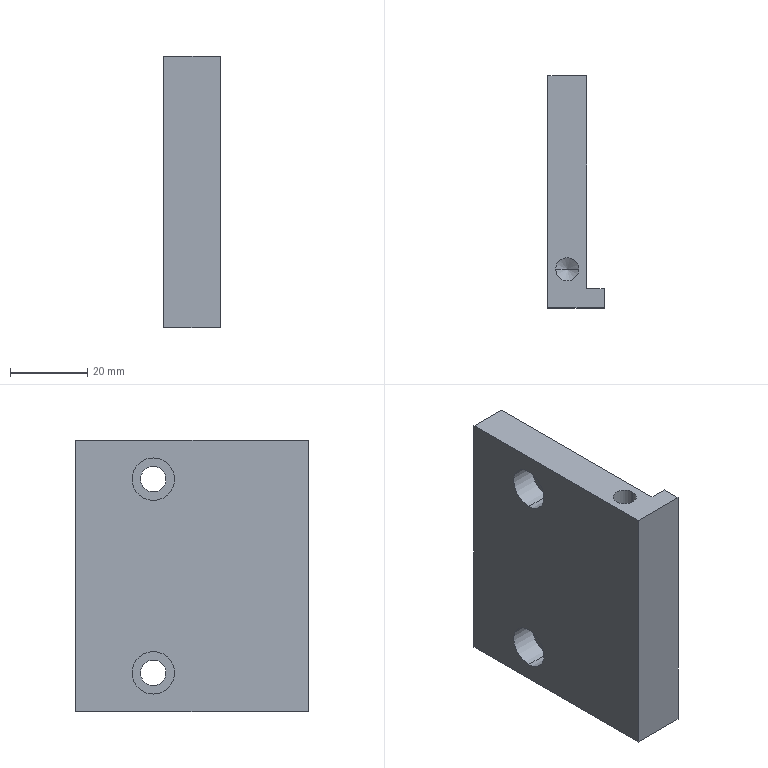Component | SolidWorks | CTM-T-12-AG-03-2 | 1 solid | 26 faces | box 14.5 x 60 x 70 mm | volume 41068 mm3 | cylinder 12 | plane 10 | cone 4 | commonest cylinder face diameters 11 x4 6.6 x4 6 x4 | material Q235A
build123d program:
from build123d import *

# Parameters (mm, degrees)
BOSS_EXTRUDE1_DEPTH                                  = 70
M6_TAPPED_HOLE1_D                                    = 6
M6_TAPPED_HOLE1_DEPTH                                = 17
M6_TAPPED_HOLE1_TIP                                  = 1.803
M6_TAPPED_HOLE2_D                                    = 6
M6_TAPPED_HOLE2_DEPTH                                = 17
M6_TAPPED_HOLE2_TIP                                  = 1.803
HOLE_SIZE_ACCORDING_TO_THE_TYPE_OF_HEXAG_D           = 6.6
HOLE_SIZE_ACCORDING_TO_THE_TYPE_OF_HEXAG_CBORE_D     = 11
HOLE_SIZE_ACCORDING_TO_THE_TYPE_OF_HEXAG_CBORE_DEPTH = 6.8


with BuildPart() as part:
    # Sketch1 → Boss-Extrude1 (new body)
    with BuildSketch(Plane.XY):
        Polygon((14.5, -5), (10, -5), (10, -60), (0, -60), (0, 0), (14.5, 0), align=None)
    extrude(amount=BOSS_EXTRUDE1_DEPTH)

    # M6 Tapped Hole1
    with Locations(Plane(origin=(0, 0, 0), x_dir=(-1, 0, 0), z_dir=(0, 0, -1))):
        with Locations((-5, -10)):
            Hole(M6_TAPPED_HOLE1_D / 2, depth=M6_TAPPED_HOLE1_DEPTH)
            with Locations((0, 0, -(M6_TAPPED_HOLE1_DEPTH + M6_TAPPED_HOLE1_TIP / 2))):  # 118° drill point
                Cone(0, M6_TAPPED_HOLE1_D / 2, M6_TAPPED_HOLE1_TIP, mode=Mode.SUBTRACT)

    # M6 Tapped Hole2
    with Locations(Plane.XY.offset(70)):
        with Locations((5, -10)):
            Hole(M6_TAPPED_HOLE2_D / 2, depth=M6_TAPPED_HOLE2_DEPTH)
            with Locations((0, 0, -(M6_TAPPED_HOLE2_DEPTH + M6_TAPPED_HOLE2_TIP / 2))):  # 118° drill point
                Cone(0, M6_TAPPED_HOLE2_D / 2, M6_TAPPED_HOLE2_TIP, mode=Mode.SUBTRACT)

    # Hole Size according to the type of Hexag (through all)
    with Locations(Plane.ZY):
        with Locations((10, -40), (60, -40)):
            CounterBoreHole(HOLE_SIZE_ACCORDING_TO_THE_TYPE_OF_HEXAG_D / 2, HOLE_SIZE_ACCORDING_TO_THE_TYPE_OF_HEXAG_CBORE_D / 2, HOLE_SIZE_ACCORDING_TO_THE_TYPE_OF_HEXAG_CBORE_DEPTH)


solid = part.part

# Placed as in the assembly
solid = solid.moved(Location((0.4, -290, 70), (180, 0, 0)))
STEP:
#1=COLOUR_RGB('',0.7922,0.8196,0.9333);
#2=FILL_AREA_STYLE_COLOUR('',#1);
#3=FILL_AREA_STYLE('',(#2));
#4=SURFACE_STYLE_FILL_AREA(#3);
#5=SURFACE_SIDE_STYLE('',(#4));
#6=SURFACE_STYLE_USAGE(.BOTH.,#5);
#7=PRESENTATION_STYLE_ASSIGNMENT((#6));
#8=CARTESIAN_POINT('',(0.2835,-9.843,2.579));
#9=VERTEX_POINT('',#8);
#10=CARTESIAN_POINT('',(0.2835,-9.843,2.146));
#11=VERTEX_POINT('',#10);
#12=CARTESIAN_POINT('',(0.2835,-9.843,2.362));
#13=DIRECTION('',(-1.,-0.,-0.));
#14=DIRECTION('',(0.,0.,-1.));
#15=AXIS2_PLACEMENT_3D('',#12,#13,#14);
#16=CIRCLE('',#15,0.2165);
#17=EDGE_CURVE('',#9,#11,#16,.T.);
#18=ORIENTED_EDGE('',*,*,#17,.F.);
#19=CARTESIAN_POINT('',(0.01575,-9.843,2.579));
#20=VERTEX_POINT('',#19);
#21=CARTESIAN_POINT('',(0.01575,-9.843,2.579));
#22=DIRECTION('',(-1.,-0.,-0.));
#23=VECTOR('',#22,39.37);
#24=LINE('',#21,#23);
#25=EDGE_CURVE('',#9,#20,#24,.T.);
#26=ORIENTED_EDGE('',*,*,#25,.T.);
#27=CARTESIAN_POINT('',(0.01575,-9.843,2.146));
#28=VERTEX_POINT('',#27);
#29=CARTESIAN_POINT('',(0.01575,-9.843,2.362));
#30=DIRECTION('',(-1.,-0.,-0.));
#31=DIRECTION('',(0.,0.,-1.));
#32=AXIS2_PLACEMENT_3D('',#29,#30,#31);
#33=CIRCLE('',#32,0.2165);
#34=EDGE_CURVE('',#20,#28,#33,.T.);
#35=ORIENTED_EDGE('',*,*,#34,.T.);
#36=CARTESIAN_POINT('',(0.01575,-9.843,2.146));
#37=DIRECTION('',(-1.,-0.,-0.));
#38=VECTOR('',#37,39.37);
#39=LINE('',#36,#38);
#40=EDGE_CURVE('',#11,#28,#39,.T.);
#41=ORIENTED_EDGE('',*,*,#40,.F.);
#42=EDGE_LOOP('',(#18,#26,#35,#41));
#43=FACE_OUTER_BOUND('',#42,.T.);
#44=CARTESIAN_POINT('',(0.01575,-9.843,2.362));
#45=DIRECTION('',(-1.,-0.,-0.));
#46=DIRECTION('',(0.,0.,-1.));
#47=AXIS2_PLACEMENT_3D('',#44,#45,#46);
#48=CYLINDRICAL_SURFACE('',#47,0.2165);
#49=ADVANCED_FACE('',(#43),#48,.F.);
#50=CARTESIAN_POINT('',(0.4094,-9.843,2.492));
#51=VERTEX_POINT('',#50);
#52=CARTESIAN_POINT('',(0.4094,-9.843,2.232));
#53=VERTEX_POINT('',#52);
#54=CARTESIAN_POINT('',(0.4094,-9.843,2.362));
#55=DIRECTION('',(-1.,-0.,-0.));
#56=DIRECTION('',(0.,1.,0.));
#57=AXIS2_PLACEMENT_3D('',#54,#55,#56);
#58=CIRCLE('',#57,0.1299);
#59=EDGE_CURVE('',#51,#53,#58,.T.);
#60=ORIENTED_EDGE('',*,*,#59,.F.);
#61=CARTESIAN_POINT('',(0.2835,-9.843,2.492));
#62=VERTEX_POINT('',#61);
#63=CARTESIAN_POINT('',(0.01575,-9.843,2.492));
#64=DIRECTION('',(-1.,-0.,-0.));
#65=VECTOR('',#64,39.37);
#66=LINE('',#63,#65);
#67=EDGE_CURVE('',#51,#62,#66,.T.);
#68=ORIENTED_EDGE('',*,*,#67,.T.);
#69=CARTESIAN_POINT('',(0.2835,-9.843,2.232));
#70=VERTEX_POINT('',#69);
#71=CARTESIAN_POINT('',(0.2835,-9.843,2.362));
#72=DIRECTION('',(-1.,-0.,-0.));
#73=DIRECTION('',(0.,0.,-1.));
#74=AXIS2_PLACEMENT_3D('',#71,#72,#73);
#75=CIRCLE('',#74,0.1299);
#76=EDGE_CURVE('',#62,#70,#75,.T.);
#77=ORIENTED_EDGE('',*,*,#76,.T.);
#78=CARTESIAN_POINT('',(0.01575,-9.843,2.232));
#79=DIRECTION('',(-1.,-0.,-0.));
#80=VECTOR('',#79,39.37);
#81=LINE('',#78,#80);
#82=EDGE_CURVE('',#53,#70,#81,.T.);
#83=ORIENTED_EDGE('',*,*,#82,.F.);
#84=EDGE_LOOP('',(#60,#68,#77,#83));
#85=FACE_OUTER_BOUND('',#84,.T.);
#86=CARTESIAN_POINT('',(0.01575,-9.843,2.362));
#87=DIRECTION('',(-1.,-0.,-0.));
#88=DIRECTION('',(0.,0.,-1.));
#89=AXIS2_PLACEMENT_3D('',#86,#87,#88);
#90=CYLINDRICAL_SURFACE('',#89,0.1299);
#91=ADVANCED_FACE('',(#85),#90,.F.);
#92=CARTESIAN_POINT('',(0.2835,-9.843,0.6102));
#93=VERTEX_POINT('',#92);
#94=CARTESIAN_POINT('',(0.2835,-9.843,0.1772));
#95=VERTEX_POINT('',#94);
#96=CARTESIAN_POINT('',(0.2835,-9.843,0.3937));
#97=DIRECTION('',(-1.,-0.,-0.));
#98=DIRECTION('',(0.,0.,-1.));
#99=AXIS2_PLACEMENT_3D('',#96,#97,#98);
#100=CIRCLE('',#99,0.2165);
#101=EDGE_CURVE('',#93,#95,#100,.T.);
#102=ORIENTED_EDGE('',*,*,#101,.F.);
#103=CARTESIAN_POINT('',(0.01575,-9.843,0.6102));
#104=VERTEX_POINT('',#103);
#105=CARTESIAN_POINT('',(0.01575,-9.843,0.6102));
#106=DIRECTION('',(-1.,-0.,-0.));
#107=VECTOR('',#106,39.37);
#108=LINE('',#105,#107);
#109=EDGE_CURVE('',#93,#104,#108,.T.);
#110=ORIENTED_EDGE('',*,*,#109,.T.);
#111=CARTESIAN_POINT('',(0.01575,-9.843,0.1772));
#112=VERTEX_POINT('',#111);
#113=CARTESIAN_POINT('',(0.01575,-9.843,0.3937));
#114=DIRECTION('',(-1.,-0.,-0.));
#115=DIRECTION('',(0.,0.,-1.));
#116=AXIS2_PLACEMENT_3D('',#113,#114,#115);
#117=CIRCLE('',#116,0.2165);
#118=EDGE_CURVE('',#104,#112,#117,.T.);
#119=ORIENTED_EDGE('',*,*,#118,.T.);
#120=CARTESIAN_POINT('',(0.01575,-9.843,0.1772));
#121=DIRECTION('',(-1.,-0.,-0.));
#122=VECTOR('',#121,39.37);
#123=LINE('',#120,#122);
#124=EDGE_CURVE('',#95,#112,#123,.T.);
#125=ORIENTED_EDGE('',*,*,#124,.F.);
#126=EDGE_LOOP('',(#102,#110,#119,#125));
#127=FACE_OUTER_BOUND('',#126,.T.);
#128=CARTESIAN_POINT('',(0.01575,-9.843,0.3937));
#129=DIRECTION('',(-1.,-0.,-0.));
#130=DIRECTION('',(0.,0.,-1.));
#131=AXIS2_PLACEMENT_3D('',#128,#129,#130);
#132=CYLINDRICAL_SURFACE('',#131,0.2165);
#133=ADVANCED_FACE('',(#127),#132,.F.);
#134=CARTESIAN_POINT('',(0.4094,-9.843,0.5236));
#135=VERTEX_POINT('',#134);
#136=CARTESIAN_POINT('',(0.4094,-9.843,0.2638));
#137=VERTEX_POINT('',#136);
#138=CARTESIAN_POINT('',(0.4094,-9.843,0.3937));
#139=DIRECTION('',(-1.,-0.,-0.));
#140=DIRECTION('',(0.,1.,-0.));
#141=AXIS2_PLACEMENT_3D('',#138,#139,#140);
#142=CIRCLE('',#141,0.1299);
#143=EDGE_CURVE('',#135,#137,#142,.T.);
#144=ORIENTED_EDGE('',*,*,#143,.F.);
#145=CARTESIAN_POINT('',(0.2835,-9.843,0.5236));
#146=VERTEX_POINT('',#145);
#147=CARTESIAN_POINT('',(0.01575,-9.843,0.5236));
#148=DIRECTION('',(-1.,-0.,-0.));
#149=VECTOR('',#148,39.37);
#150=LINE('',#147,#149);
#151=EDGE_CURVE('',#135,#146,#150,.T.);
#152=ORIENTED_EDGE('',*,*,#151,.T.);
#153=CARTESIAN_POINT('',(0.2835,-9.843,0.2638));
#154=VERTEX_POINT('',#153);
#155=CARTESIAN_POINT('',(0.2835,-9.843,0.3937));
#156=DIRECTION('',(-1.,-0.,-0.));
#157=DIRECTION('',(0.,0.,-1.));
#158=AXIS2_PLACEMENT_3D('',#155,#156,#157);
#159=CIRCLE('',#158,0.1299);
#160=EDGE_CURVE('',#146,#154,#159,.T.);
#161=ORIENTED_EDGE('',*,*,#160,.T.);
#162=CARTESIAN_POINT('',(0.01575,-9.843,0.2638));
#163=DIRECTION('',(-1.,-0.,-0.));
#164=VECTOR('',#163,39.37);
#165=LINE('',#162,#164);
#166=EDGE_CURVE('',#137,#154,#165,.T.);
#167=ORIENTED_EDGE('',*,*,#166,.F.);
#168=EDGE_LOOP('',(#144,#152,#161,#167));
#169=FACE_OUTER_BOUND('',#168,.T.);
#170=CARTESIAN_POINT('',(0.01575,-9.843,0.3937));
#171=DIRECTION('',(-1.,-0.,-0.));
#172=DIRECTION('',(0.,0.,-1.));
#173=AXIS2_PLACEMENT_3D('',#170,#171,#172);
#174=CYLINDRICAL_SURFACE('',#173,0.1299);
#175=ADVANCED_FACE('',(#169),#174,.F.);
#176=CARTESIAN_POINT('',(0.09449,-11.024,0.6693));
#177=VERTEX_POINT('',#176);
#178=CARTESIAN_POINT('',(0.3307,-11.024,0.6693));
#179=VERTEX_POINT('',#178);
#180=CARTESIAN_POINT('',(0.2126,-11.024,0.6693));
#181=DIRECTION('',(0.,-0.,-1.));
#182=DIRECTION('',(1.,0.,0.));
#183=AXIS2_PLACEMENT_3D('',#180,#181,#182);
#184=CIRCLE('',#183,0.1181);
#185=EDGE_CURVE('',#177,#179,#184,.T.);
#186=ORIENTED_EDGE('',*,*,#185,.F.);
#187=CARTESIAN_POINT('',(0.09449,-11.024,-0.));
#188=VERTEX_POINT('',#187);
#189=CARTESIAN_POINT('',(0.09449,-11.024,-0.));
#190=DIRECTION('',(0.,-0.,-1.));
#191=VECTOR('',#190,39.37);
#192=LINE('',#189,#191);
#193=EDGE_CURVE('',#177,#188,#192,.T.);
#194=ORIENTED_EDGE('',*,*,#193,.T.);
#195=CARTESIAN_POINT('',(0.3307,-11.024,-0.));
#196=VERTEX_POINT('',#195);
#197=CARTESIAN_POINT('',(0.2126,-11.024,-0.));
#198=DIRECTION('',(0.,-0.,-1.));
#199=DIRECTION('',(1.,0.,0.));
#200=AXIS2_PLACEMENT_3D('',#197,#198,#199);
#201=CIRCLE('',#200,0.1181);
#202=EDGE_CURVE('',#188,#196,#201,.T.);
#203=ORIENTED_EDGE('',*,*,#202,.T.);
#204=CARTESIAN_POINT('',(0.3307,-11.024,-0.));
#205=DIRECTION('',(0.,-0.,-1.));
#206=VECTOR('',#205,39.37);
#207=LINE('',#204,#206);
#208=EDGE_CURVE('',#179,#196,#207,.T.);
#209=ORIENTED_EDGE('',*,*,#208,.F.);
#210=EDGE_LOOP('',(#186,#194,#203,#209));
#211=FACE_OUTER_BOUND('',#210,.T.);
#212=CARTESIAN_POINT('',(0.2126,-11.024,-0.));
#213=DIRECTION('',(0.,-0.,-1.));
#214=DIRECTION('',(1.,0.,0.));
#215=AXIS2_PLACEMENT_3D('',#212,#213,#214);
#216=CYLINDRICAL_SURFACE('',#215,0.1181);
#217=ADVANCED_FACE('',(#211),#216,.F.);
#218=CARTESIAN_POINT('',(0.2126,-11.024,0.7403));
#219=VERTEX_POINT('',#218);
#220=CARTESIAN_POINT('',(0.3307,-11.024,0.6693));
#221=DIRECTION('',(0.8572,-0.,-0.515));
#222=VECTOR('',#221,39.37);
#223=LINE('',#220,#222);
#224=EDGE_CURVE('',#219,#179,#223,.T.);
#225=ORIENTED_EDGE('',*,*,#224,.F.);
#226=CARTESIAN_POINT('',(0.09449,-11.024,0.6693));
#227=DIRECTION('',(-0.8572,-0.,-0.515));
#228=VECTOR('',#227,39.37);
#229=LINE('',#226,#228);
#230=EDGE_CURVE('',#219,#177,#229,.T.);
#231=ORIENTED_EDGE('',*,*,#230,.T.);
#232=ORIENTED_EDGE('',*,*,#185,.T.);
#233=EDGE_LOOP('',(#225,#231,#232));
#234=FACE_OUTER_BOUND('',#233,.T.);
#235=CARTESIAN_POINT('',(0.2126,-11.024,0.6693));
#236=DIRECTION('',(0.,-0.,-1.));
#237=DIRECTION('',(1.,0.,0.));
#238=AXIS2_PLACEMENT_3D('',#235,#236,#237);
#239=CONICAL_SURFACE('',#238,0.1181,1.03);
#240=ADVANCED_FACE('',(#234),#239,.F.);
#241=CARTESIAN_POINT('',(0.3307,-11.024,2.087));
#242=VERTEX_POINT('',#241);
#243=CARTESIAN_POINT('',(0.09449,-11.024,2.087));
#244=VERTEX_POINT('',#243);
#245=CARTESIAN_POINT('',(0.2126,-11.024,2.087));
#246=DIRECTION('',(-0.,0.,1.));
#247=DIRECTION('',(-1.,0.,0.));
#248=AXIS2_PLACEMENT_3D('',#245,#246,#247);
#249=CIRCLE('',#248,0.1181);
#250=EDGE_CURVE('',#242,#244,#249,.T.);
#251=ORIENTED_EDGE('',*,*,#250,.F.);
#252=CARTESIAN_POINT('',(0.3307,-11.024,2.756));
#253=VERTEX_POINT('',#252);
#254=CARTESIAN_POINT('',(0.3307,-11.024,2.756));
#255=DIRECTION('',(-0.,0.,1.));
#256=VECTOR('',#255,39.37);
#257=LINE('',#254,#256);
#258=EDGE_CURVE('',#242,#253,#257,.T.);
#259=ORIENTED_EDGE('',*,*,#258,.T.);
#260=CARTESIAN_POINT('',(0.09449,-11.024,2.756));
#261=VERTEX_POINT('',#260);
#262=CARTESIAN_POINT('',(0.2126,-11.024,2.756));
#263=DIRECTION('',(-0.,0.,1.));
#264=DIRECTION('',(-1.,0.,0.));
#265=AXIS2_PLACEMENT_3D('',#262,#263,#264);
#266=CIRCLE('',#265,0.1181);
#267=EDGE_CURVE('',#253,#261,#266,.T.);
#268=ORIENTED_EDGE('',*,*,#267,.T.);
#269=CARTESIAN_POINT('',(0.09449,-11.024,2.756));
#270=DIRECTION('',(-0.,0.,1.));
#271=VECTOR('',#270,39.37);
#272=LINE('',#269,#271);
#273=EDGE_CURVE('',#244,#261,#272,.T.);
#274=ORIENTED_EDGE('',*,*,#273,.F.);
#275=EDGE_LOOP('',(#251,#259,#268,#274));
#276=FACE_OUTER_BOUND('',#275,.T.);
#277=CARTESIAN_POINT('',(0.2126,-11.024,2.756));
#278=DIRECTION('',(-0.,0.,1.));
#279=DIRECTION('',(-1.,0.,0.));
#280=AXIS2_PLACEMENT_3D('',#277,#278,#279);
#281=CYLINDRICAL_SURFACE('',#280,0.1181);
#282=ADVANCED_FACE('',(#276),#281,.F.);
#283=CARTESIAN_POINT('',(0.2126,-11.024,2.016));
#284=VERTEX_POINT('',#283);
#285=CARTESIAN_POINT('',(0.09449,-11.024,2.087));
#286=DIRECTION('',(-0.8572,0.,0.515));
#287=VECTOR('',#286,39.37);
#288=LINE('',#285,#287);
#289=EDGE_CURVE('',#284,#244,#288,.T.);
#290=ORIENTED_EDGE('',*,*,#289,.F.);
#291=CARTESIAN_POINT('',(0.3307,-11.024,2.087));
#292=DIRECTION('',(0.8572,0.,0.515));
#293=VECTOR('',#292,39.37);
#294=LINE('',#291,#293);
#295=EDGE_CURVE('',#284,#242,#294,.T.);
#296=ORIENTED_EDGE('',*,*,#295,.T.);
#297=ORIENTED_EDGE('',*,*,#250,.T.);
#298=EDGE_LOOP('',(#290,#296,#297));
#299=FACE_OUTER_BOUND('',#298,.T.);
#300=CARTESIAN_POINT('',(0.2126,-11.024,2.087));
#301=DIRECTION('',(-0.,0.,1.));
#302=DIRECTION('',(-1.,0.,0.));
#303=AXIS2_PLACEMENT_3D('',#300,#301,#302);
#304=CONICAL_SURFACE('',#303,0.1181,1.03);
#305=ADVANCED_FACE('',(#299),#304,.F.);
#306=CARTESIAN_POINT('',(0.01575,-9.843,2.362));
#307=DIRECTION('',(-1.,-0.,-0.));
#308=DIRECTION('',(0.,0.,-1.));
#309=AXIS2_PLACEMENT_3D('',#306,#307,#308);
#310=CIRCLE('',#309,0.2165);
#311=EDGE_CURVE('',#28,#20,#310,.T.);
#312=ORIENTED_EDGE('',*,*,#311,.F.);
#313=ORIENTED_EDGE('',*,*,#34,.F.);
#314=EDGE_LOOP('',(#312,#313));
#315=FACE_BOUND('',#314,.T.);
#316=CARTESIAN_POINT('',(0.01575,-9.843,0.3937));
#317=DIRECTION('',(-1.,-0.,-0.));
#318=DIRECTION('',(0.,0.,-1.));
#319=AXIS2_PLACEMENT_3D('',#316,#317,#318);
#320=CIRCLE('',#319,0.2165);
#321=EDGE_CURVE('',#112,#104,#320,.T.);
#322=ORIENTED_EDGE('',*,*,#321,.F.);
#323=ORIENTED_EDGE('',*,*,#118,.F.);
#324=EDGE_LOOP('',(#322,#323));
#325=FACE_BOUND('',#324,.T.);
#326=CARTESIAN_POINT('',(0.01575,-11.417,2.756));
#327=VERTEX_POINT('',#326);
#328=CARTESIAN_POINT('',(0.01575,-9.055,2.756));
#329=VERTEX_POINT('',#328);
#330=CARTESIAN_POINT('',(0.01575,-11.417,2.756));
#331=DIRECTION('',(-0.,1.,-0.));
#332=VECTOR('',#331,39.37);
#333=LINE('',#330,#332);
#334=EDGE_CURVE('',#327,#329,#333,.T.);
#335=ORIENTED_EDGE('',*,*,#334,.T.);
#336=CARTESIAN_POINT('',(0.01575,-9.055,-0.));
#337=VERTEX_POINT('',#336);
#338=CARTESIAN_POINT('',(0.01575,-9.055,-0.));
#339=DIRECTION('',(-0.,0.,1.));
#340=VECTOR('',#339,39.37);
#341=LINE('',#338,#340);
#342=EDGE_CURVE('',#337,#329,#341,.T.);
#343=ORIENTED_EDGE('',*,*,#342,.F.);
#344=CARTESIAN_POINT('',(0.01575,-11.417,-0.));
#345=VERTEX_POINT('',#344);
#346=CARTESIAN_POINT('',(0.01575,-11.417,-0.));
#347=DIRECTION('',(-0.,1.,-0.));
#348=VECTOR('',#347,39.37);
#349=LINE('',#346,#348);
#350=EDGE_CURVE('',#345,#337,#349,.T.);
#351=ORIENTED_EDGE('',*,*,#350,.F.);
#352=CARTESIAN_POINT('',(0.01575,-11.417,-0.));
#353=DIRECTION('',(-0.,0.,1.));
#354=VECTOR('',#353,39.37);
#355=LINE('',#352,#354);
#356=EDGE_CURVE('',#345,#327,#355,.T.);
#357=ORIENTED_EDGE('',*,*,#356,.T.);
#358=EDGE_LOOP('',(#335,#343,#351,#357));
#359=FACE_OUTER_BOUND('',#358,.T.);
#360=CARTESIAN_POINT('',(0.01575,-11.417,-0.));
#361=DIRECTION('',(1.,0.,0.));
#362=DIRECTION('',(0.,-1.,0.));
#363=AXIS2_PLACEMENT_3D('',#360,#361,#362);
#364=PLANE('',#363);
#365=ADVANCED_FACE('',(#315,#325,#359),#364,.F.);
#366=CARTESIAN_POINT('',(0.4094,-9.055,2.756));
#367=VERTEX_POINT('',#366);
#368=CARTESIAN_POINT('',(0.01575,-9.055,2.756));
#369=DIRECTION('',(1.,0.,0.));
#370=VECTOR('',#369,39.37);
#371=LINE('',#368,#370);
#372=EDGE_CURVE('',#329,#367,#371,.T.);
#373=ORIENTED_EDGE('',*,*,#372,.T.);
#374=CARTESIAN_POINT('',(0.4094,-9.055,-0.));
#375=VERTEX_POINT('',#374);
#376=CARTESIAN_POINT('',(0.4094,-9.055,-0.));
#377=DIRECTION('',(-0.,0.,1.));
#378=VECTOR('',#377,39.37);
#379=LINE('',#376,#378);
#380=EDGE_CURVE('',#375,#367,#379,.T.);
#381=ORIENTED_EDGE('',*,*,#380,.F.);
#382=CARTESIAN_POINT('',(0.01575,-9.055,-0.));
#383=DIRECTION('',(1.,0.,0.));
#384=VECTOR('',#383,39.37);
#385=LINE('',#382,#384);
#386=EDGE_CURVE('',#337,#375,#385,.T.);
#387=ORIENTED_EDGE('',*,*,#386,.F.);
#388=ORIENTED_EDGE('',*,*,#342,.T.);
#389=EDGE_LOOP('',(#373,#381,#387,#388));
#390=FACE_OUTER_BOUND('',#389,.T.);
#391=CARTESIAN_POINT('',(0.01575,-9.055,-0.));
#392=DIRECTION('',(0.,-1.,0.));
#393=DIRECTION('',(0.,-0.,-1.));
#394=AXIS2_PLACEMENT_3D('',#391,#392,#393);
#395=PLANE('',#394);
#396=ADVANCED_FACE('',(#390),#395,.F.);
#397=CARTESIAN_POINT('',(0.4094,-9.843,2.362));
#398=DIRECTION('',(-1.,-0.,-0.));
#399=DIRECTION('',(0.,1.,0.));
#400=AXIS2_PLACEMENT_3D('',#397,#398,#399);
#401=CIRCLE('',#400,0.1299);
#402=EDGE_CURVE('',#53,#51,#401,.T.);
#403=ORIENTED_EDGE('',*,*,#402,.T.);
#404=ORIENTED_EDGE('',*,*,#59,.T.);
#405=EDGE_LOOP('',(#403,#404));
#406=FACE_BOUND('',#405,.T.);
#407=CARTESIAN_POINT('',(0.4094,-9.843,0.3937));
#408=DIRECTION('',(-1.,-0.,-0.));
#409=DIRECTION('',(0.,1.,-0.));
#410=AXIS2_PLACEMENT_3D('',#407,#408,#409);
#411=CIRCLE('',#410,0.1299);
#412=EDGE_CURVE('',#137,#135,#411,.T.);
#413=ORIENTED_EDGE('',*,*,#412,.T.);
#414=ORIENTED_EDGE('',*,*,#143,.T.);
#415=EDGE_LOOP('',(#413,#414));
#416=FACE_BOUND('',#415,.T.);
#417=CARTESIAN_POINT('',(0.4094,-11.22,2.756));
#418=VERTEX_POINT('',#417);
#419=CARTESIAN_POINT('',(0.4094,-11.22,2.756));
#420=DIRECTION('',(0.,-1.,0.));
#421=VECTOR('',#420,39.37);
#422=LINE('',#419,#421);
#423=EDGE_CURVE('',#367,#418,#422,.T.);
#424=ORIENTED_EDGE('',*,*,#423,.T.);
#425=CARTESIAN_POINT('',(0.4094,-11.22,-0.));
#426=VERTEX_POINT('',#425);
#427=CARTESIAN_POINT('',(0.4094,-11.22,-0.));
#428=DIRECTION('',(-0.,0.,1.));
#429=VECTOR('',#428,39.37);
#430=LINE('',#427,#429);
#431=EDGE_CURVE('',#426,#418,#430,.T.);
#432=ORIENTED_EDGE('',*,*,#431,.F.);
#433=CARTESIAN_POINT('',(0.4094,-11.22,-0.));
#434=DIRECTION('',(0.,-1.,0.));
#435=VECTOR('',#434,39.37);
#436=LINE('',#433,#435);
#437=EDGE_CURVE('',#375,#426,#436,.T.);
#438=ORIENTED_EDGE('',*,*,#437,.F.);
#439=ORIENTED_EDGE('',*,*,#380,.T.);
#440=EDGE_LOOP('',(#424,#432,#438,#439));
#441=FACE_OUTER_BOUND('',#440,.T.);
#442=CARTESIAN_POINT('',(0.4094,-11.22,-0.));
#443=DIRECTION('',(-1.,-0.,-0.));
#444=DIRECTION('',(-0.,1.,-0.));
#445=AXIS2_PLACEMENT_3D('',#442,#443,#444);
#446=PLANE('',#445);
#447=ADVANCED_FACE('',(#406,#416,#441),#446,.F.);
#448=CARTESIAN_POINT('',(0.5866,-11.22,2.756));
#449=VERTEX_POINT('',#448);
#450=CARTESIAN_POINT('',(0.5866,-11.22,2.756));
#451=DIRECTION('',(1.,0.,0.));
#452=VECTOR('',#451,39.37);
#453=LINE('',#450,#452);
#454=EDGE_CURVE('',#418,#449,#453,.T.);
#455=ORIENTED_EDGE('',*,*,#454,.T.);
#456=CARTESIAN_POINT('',(0.5866,-11.22,-0.));
#457=VERTEX_POINT('',#456);
#458=CARTESIAN_POINT('',(0.5866,-11.22,-0.));
#459=DIRECTION('',(-0.,0.,1.));
#460=VECTOR('',#459,39.37);
#461=LINE('',#458,#460);
#462=EDGE_CURVE('',#457,#449,#461,.T.);
#463=ORIENTED_EDGE('',*,*,#462,.F.);
#464=CARTESIAN_POINT('',(0.5866,-11.22,-0.));
#465=DIRECTION('',(1.,0.,0.));
#466=VECTOR('',#465,39.37);
#467=LINE('',#464,#466);
#468=EDGE_CURVE('',#426,#457,#467,.T.);
#469=ORIENTED_EDGE('',*,*,#468,.F.);
#470=ORIENTED_EDGE('',*,*,#431,.T.);
#471=EDGE_LOOP('',(#455,#463,#469,#470));
#472=FACE_OUTER_BOUND('',#471,.T.);
#473=CARTESIAN_POINT('',(0.5866,-11.22,-0.));
#474=DIRECTION('',(0.,-1.,0.));
#475=DIRECTION('',(0.,-0.,-1.));
#476=AXIS2_PLACEMENT_3D('',#473,#474,#475);
#477=PLANE('',#476);
#478=ADVANCED_FACE('',(#472),#477,.F.);
#479=CARTESIAN_POINT('',(0.5866,-11.417,2.756));
#480=VERTEX_POINT('',#479);
#481=CARTESIAN_POINT('',(0.5866,-11.417,2.756));
#482=DIRECTION('',(0.,-1.,0.));
#483=VECTOR('',#482,39.37);
#484=LINE('',#481,#483);
#485=EDGE_CURVE('',#449,#480,#484,.T.);
#486=ORIENTED_EDGE('',*,*,#485,.T.);
#487=CARTESIAN_POINT('',(0.5866,-11.417,-0.));
#488=VERTEX_POINT('',#487);
#489=CARTESIAN_POINT('',(0.5866,-11.417,-0.));
#490=DIRECTION('',(-0.,0.,1.));
#491=VECTOR('',#490,39.37);
#492=LINE('',#489,#491);
#493=EDGE_CURVE('',#488,#480,#492,.T.);
#494=ORIENTED_EDGE('',*,*,#493,.F.);
#495=CARTESIAN_POINT('',(0.5866,-11.417,-0.));
#496=DIRECTION('',(0.,-1.,0.));
#497=VECTOR('',#496,39.37);
#498=LINE('',#495,#497);
#499=EDGE_CURVE('',#457,#488,#498,.T.);
#500=ORIENTED_EDGE('',*,*,#499,.F.);
#501=ORIENTED_EDGE('',*,*,#462,.T.);
#502=EDGE_LOOP('',(#486,#494,#500,#501));
#503=FACE_OUTER_BOUND('',#502,.T.);
#504=CARTESIAN_POINT('',(0.5866,-11.417,-0.));
#505=DIRECTION('',(-1.,-0.,-0.));
#506=DIRECTION('',(0.,-0.,-1.));
#507=AXIS2_PLACEMENT_3D('',#504,#505,#506);
#508=PLANE('',#507);
#509=ADVANCED_FACE('',(#503),#508,.F.);
#510=CARTESIAN_POINT('',(0.01575,-11.417,2.756));
#511=DIRECTION('',(-1.,-0.,-0.));
#512=VECTOR('',#511,39.37);
#513=LINE('',#510,#512);
#514=EDGE_CURVE('',#480,#327,#513,.T.);
#515=ORIENTED_EDGE('',*,*,#514,.T.);
#516=ORIENTED_EDGE('',*,*,#356,.F.);
#517=CARTESIAN_POINT('',(0.01575,-11.417,-0.));
#518=DIRECTION('',(-1.,-0.,-0.));
#519=VECTOR('',#518,39.37);
#520=LINE('',#517,#519);
#521=EDGE_CURVE('',#488,#345,#520,.T.);
#522=ORIENTED_EDGE('',*,*,#521,.F.);
#523=ORIENTED_EDGE('',*,*,#493,.T.);
#524=EDGE_LOOP('',(#515,#516,#522,#523));
#525=FACE_OUTER_BOUND('',#524,.T.);
#526=CARTESIAN_POINT('',(0.01575,-11.417,-0.));
#527=DIRECTION('',(-0.,1.,-0.));
#528=DIRECTION('',(-0.,0.,1.));
#529=AXIS2_PLACEMENT_3D('',#526,#527,#528);
#530=PLANE('',#529);
#531=ADVANCED_FACE('',(#525),#530,.F.);
#532=CARTESIAN_POINT('',(0.2126,-11.024,-0.));
#533=DIRECTION('',(0.,-0.,-1.));
#534=DIRECTION('',(1.,0.,0.));
#535=AXIS2_PLACEMENT_3D('',#532,#533,#534);
#536=CIRCLE('',#535,0.1181);
#537=EDGE_CURVE('',#196,#188,#536,.T.);
#538=ORIENTED_EDGE('',*,*,#537,.F.);
#539=ORIENTED_EDGE('',*,*,#202,.F.);
#540=EDGE_LOOP('',(#538,#539));
#541=FACE_BOUND('',#540,.T.);
#542=ORIENTED_EDGE('',*,*,#350,.T.);
#543=ORIENTED_EDGE('',*,*,#386,.T.);
#544=ORIENTED_EDGE('',*,*,#437,.T.);
#545=ORIENTED_EDGE('',*,*,#468,.T.);
#546=ORIENTED_EDGE('',*,*,#499,.T.);
#547=ORIENTED_EDGE('',*,*,#521,.T.);
#548=EDGE_LOOP('',(#542,#543,#544,#545,#546,#547));
#549=FACE_OUTER_BOUND('',#548,.T.);
#550=CARTESIAN_POINT('',(0.01575,-9.055,-0.));
#551=DIRECTION('',(0.,-0.,-1.));
#552=DIRECTION('',(1.,0.,0.));
#553=AXIS2_PLACEMENT_3D('',#550,#551,#552);
#554=PLANE('',#553);
#555=ADVANCED_FACE('',(#541,#549),#554,.T.);
#556=CARTESIAN_POINT('',(0.2126,-11.024,2.756));
#557=DIRECTION('',(-0.,0.,1.));
#558=DIRECTION('',(-1.,0.,0.));
#559=AXIS2_PLACEMENT_3D('',#556,#557,#558);
#560=CIRCLE('',#559,0.1181);
#561=EDGE_CURVE('',#261,#253,#560,.T.);
#562=ORIENTED_EDGE('',*,*,#561,.F.);
#563=ORIENTED_EDGE('',*,*,#267,.F.);
#564=EDGE_LOOP('',(#562,#563));
#565=FACE_BOUND('',#564,.T.);
#566=ORIENTED_EDGE('',*,*,#334,.F.);
#567=ORIENTED_EDGE('',*,*,#514,.F.);
#568=ORIENTED_EDGE('',*,*,#485,.F.);
#569=ORIENTED_EDGE('',*,*,#454,.F.);
#570=ORIENTED_EDGE('',*,*,#423,.F.);
#571=ORIENTED_EDGE('',*,*,#372,.F.);
#572=EDGE_LOOP('',(#566,#567,#568,#569,#570,#571));
#573=FACE_OUTER_BOUND('',#572,.T.);
#574=CARTESIAN_POINT('',(0.01575,-9.055,2.756));
#575=DIRECTION('',(0.,-0.,-1.));
#576=DIRECTION('',(1.,0.,0.));
#577=AXIS2_PLACEMENT_3D('',#574,#575,#576);
#578=PLANE('',#577);
#579=ADVANCED_FACE('',(#565,#573),#578,.F.);
#580=ORIENTED_EDGE('',*,*,#295,.F.);
#581=ORIENTED_EDGE('',*,*,#289,.T.);
#582=CARTESIAN_POINT('',(0.2126,-11.024,2.087));
#583=DIRECTION('',(-0.,0.,1.));
#584=DIRECTION('',(-1.,0.,0.));
#585=AXIS2_PLACEMENT_3D('',#582,#583,#584);
#586=CIRCLE('',#585,0.1181);
#587=EDGE_CURVE('',#244,#242,#586,.T.);
#588=ORIENTED_EDGE('',*,*,#587,.T.);
#589=EDGE_LOOP('',(#580,#581,#588));
#590=FACE_OUTER_BOUND('',#589,.T.);
#591=CARTESIAN_POINT('',(0.2126,-11.024,2.087));
#592=DIRECTION('',(-0.,0.,1.));
#593=DIRECTION('',(-1.,0.,0.));
#594=AXIS2_PLACEMENT_3D('',#591,#592,#593);
#595=CONICAL_SURFACE('',#594,0.1181,1.03);
#596=ADVANCED_FACE('',(#590),#595,.F.);
#597=ORIENTED_EDGE('',*,*,#258,.F.);
#598=ORIENTED_EDGE('',*,*,#587,.F.);
#599=ORIENTED_EDGE('',*,*,#273,.T.);
#600=ORIENTED_EDGE('',*,*,#561,.T.);
#601=EDGE_LOOP('',(#597,#598,#599,#600));
#602=FACE_OUTER_BOUND('',#601,.T.);
#603=CARTESIAN_POINT('',(0.2126,-11.024,2.756));
#604=DIRECTION('',(-0.,0.,1.));
#605=DIRECTION('',(-1.,0.,0.));
#606=AXIS2_PLACEMENT_3D('',#603,#604,#605);
#607=CYLINDRICAL_SURFACE('',#606,0.1181);
#608=ADVANCED_FACE('',(#602),#607,.F.);
#609=ORIENTED_EDGE('',*,*,#230,.F.);
#610=ORIENTED_EDGE('',*,*,#224,.T.);
#611=CARTESIAN_POINT('',(0.2126,-11.024,0.6693));
#612=DIRECTION('',(0.,-0.,-1.));
#613=DIRECTION('',(1.,0.,0.));
#614=AXIS2_PLACEMENT_3D('',#611,#612,#613);
#615=CIRCLE('',#614,0.1181);
#616=EDGE_CURVE('',#179,#177,#615,.T.);
#617=ORIENTED_EDGE('',*,*,#616,.T.);
#618=EDGE_LOOP('',(#609,#610,#617));
#619=FACE_OUTER_BOUND('',#618,.T.);
#620=CARTESIAN_POINT('',(0.2126,-11.024,0.6693));
#621=DIRECTION('',(0.,-0.,-1.));
#622=DIRECTION('',(1.,0.,0.));
#623=AXIS2_PLACEMENT_3D('',#620,#621,#622);
#624=CONICAL_SURFACE('',#623,0.1181,1.03);
#625=ADVANCED_FACE('',(#619),#624,.F.);
#626=ORIENTED_EDGE('',*,*,#193,.F.);
#627=ORIENTED_EDGE('',*,*,#616,.F.);
#628=ORIENTED_EDGE('',*,*,#208,.T.);
#629=ORIENTED_EDGE('',*,*,#537,.T.);
#630=EDGE_LOOP('',(#626,#627,#628,#629));
#631=FACE_OUTER_BOUND('',#630,.T.);
#632=CARTESIAN_POINT('',(0.2126,-11.024,-0.));
#633=DIRECTION('',(0.,-0.,-1.));
#634=DIRECTION('',(1.,0.,0.));
#635=AXIS2_PLACEMENT_3D('',#632,#633,#634);
#636=CYLINDRICAL_SURFACE('',#635,0.1181);
#637=ADVANCED_FACE('',(#631),#636,.F.);
#638=ORIENTED_EDGE('',*,*,#151,.F.);
#639=ORIENTED_EDGE('',*,*,#412,.F.);
#640=ORIENTED_EDGE('',*,*,#166,.T.);
#641=CARTESIAN_POINT('',(0.2835,-9.843,0.3937));
#642=DIRECTION('',(-1.,-0.,-0.));
#643=DIRECTION('',(0.,0.,-1.));
#644=AXIS2_PLACEMENT_3D('',#641,#642,#643);
#645=CIRCLE('',#644,0.1299);
#646=EDGE_CURVE('',#154,#146,#645,.T.);
#647=ORIENTED_EDGE('',*,*,#646,.T.);
#648=EDGE_LOOP('',(#638,#639,#640,#647));
#649=FACE_OUTER_BOUND('',#648,.T.);
#650=CARTESIAN_POINT('',(0.01575,-9.843,0.3937));
#651=DIRECTION('',(-1.,-0.,-0.));
#652=DIRECTION('',(0.,0.,-1.));
#653=AXIS2_PLACEMENT_3D('',#650,#651,#652);
#654=CYLINDRICAL_SURFACE('',#653,0.1299);
#655=ADVANCED_FACE('',(#649),#654,.F.);
#656=ORIENTED_EDGE('',*,*,#646,.F.);
#657=ORIENTED_EDGE('',*,*,#160,.F.);
#658=EDGE_LOOP('',(#656,#657));
#659=FACE_BOUND('',#658,.T.);
#660=CARTESIAN_POINT('',(0.2835,-9.843,0.3937));
#661=DIRECTION('',(-1.,-0.,-0.));
#662=DIRECTION('',(0.,0.,-1.));
#663=AXIS2_PLACEMENT_3D('',#660,#661,#662);
#664=CIRCLE('',#663,0.2165);
#665=EDGE_CURVE('',#95,#93,#664,.T.);
#666=ORIENTED_EDGE('',*,*,#665,.T.);
#667=ORIENTED_EDGE('',*,*,#101,.T.);
#668=EDGE_LOOP('',(#666,#667));
#669=FACE_OUTER_BOUND('',#668,.T.);
#670=CARTESIAN_POINT('',(0.2835,-9.972,0.3937));
#671=DIRECTION('',(1.,0.,0.));
#672=DIRECTION('',(-0.,0.,1.));
#673=AXIS2_PLACEMENT_3D('',#670,#671,#672);
#674=PLANE('',#673);
#675=ADVANCED_FACE('',(#659,#669),#674,.F.);
#676=ORIENTED_EDGE('',*,*,#109,.F.);
#677=ORIENTED_EDGE('',*,*,#665,.F.);
#678=ORIENTED_EDGE('',*,*,#124,.T.);
#679=ORIENTED_EDGE('',*,*,#321,.T.);
#680=EDGE_LOOP('',(#676,#677,#678,#679));
#681=FACE_OUTER_BOUND('',#680,.T.);
#682=CARTESIAN_POINT('',(0.01575,-9.843,0.3937));
#683=DIRECTION('',(-1.,-0.,-0.));
#684=DIRECTION('',(0.,0.,-1.));
#685=AXIS2_PLACEMENT_3D('',#682,#683,#684);
#686=CYLINDRICAL_SURFACE('',#685,0.2165);
#687=ADVANCED_FACE('',(#681),#686,.F.);
#688=ORIENTED_EDGE('',*,*,#67,.F.);
#689=ORIENTED_EDGE('',*,*,#402,.F.);
#690=ORIENTED_EDGE('',*,*,#82,.T.);
#691=CARTESIAN_POINT('',(0.2835,-9.843,2.362));
#692=DIRECTION('',(-1.,-0.,-0.));
#693=DIRECTION('',(0.,0.,-1.));
#694=AXIS2_PLACEMENT_3D('',#691,#692,#693);
#695=CIRCLE('',#694,0.1299);
#696=EDGE_CURVE('',#70,#62,#695,.T.);
#697=ORIENTED_EDGE('',*,*,#696,.T.);
#698=EDGE_LOOP('',(#688,#689,#690,#697));
#699=FACE_OUTER_BOUND('',#698,.T.);
#700=CARTESIAN_POINT('',(0.01575,-9.843,2.362));
#701=DIRECTION('',(-1.,-0.,-0.));
#702=DIRECTION('',(0.,0.,-1.));
#703=AXIS2_PLACEMENT_3D('',#700,#701,#702);
#704=CYLINDRICAL_SURFACE('',#703,0.1299);
#705=ADVANCED_FACE('',(#699),#704,.F.);
#706=ORIENTED_EDGE('',*,*,#696,.F.);
#707=ORIENTED_EDGE('',*,*,#76,.F.);
#708=EDGE_LOOP('',(#706,#707));
#709=FACE_BOUND('',#708,.T.);
#710=CARTESIAN_POINT('',(0.2835,-9.843,2.362));
#711=DIRECTION('',(-1.,-0.,-0.));
#712=DIRECTION('',(0.,0.,-1.));
#713=AXIS2_PLACEMENT_3D('',#710,#711,#712);
#714=CIRCLE('',#713,0.2165);
#715=EDGE_CURVE('',#11,#9,#714,.T.);
#716=ORIENTED_EDGE('',*,*,#715,.T.);
#717=ORIENTED_EDGE('',*,*,#17,.T.);
#718=EDGE_LOOP('',(#716,#717));
#719=FACE_OUTER_BOUND('',#718,.T.);
#720=CARTESIAN_POINT('',(0.2835,-9.972,2.362));
#721=DIRECTION('',(1.,0.,0.));
#722=DIRECTION('',(-0.,0.,1.));
#723=AXIS2_PLACEMENT_3D('',#720,#721,#722);
#724=PLANE('',#723);
#725=ADVANCED_FACE('',(#709,#719),#724,.F.);
#726=ORIENTED_EDGE('',*,*,#25,.F.);
#727=ORIENTED_EDGE('',*,*,#715,.F.);
#728=ORIENTED_EDGE('',*,*,#40,.T.);
#729=ORIENTED_EDGE('',*,*,#311,.T.);
#730=EDGE_LOOP('',(#726,#727,#728,#729));
#731=FACE_OUTER_BOUND('',#730,.T.);
#732=CARTESIAN_POINT('',(0.01575,-9.843,2.362));
#733=DIRECTION('',(-1.,-0.,-0.));
#734=DIRECTION('',(0.,0.,-1.));
#735=AXIS2_PLACEMENT_3D('',#732,#733,#734);
#736=CYLINDRICAL_SURFACE('',#735,0.2165);
#737=ADVANCED_FACE('',(#731),#736,.F.);
#738=CLOSED_SHELL('',(#49,#91,#133,#175,#217,#240,#282,#305,#365,#396,#447,#478,#509,#531,#555,#579,#596,#608,#625,#637,#655,#675,#687,#705,#725,#737));
#739=MANIFOLD_SOLID_BREP('',#738);
#740=STYLED_ITEM('',(#7),#739);
#741=PRESENTATION_LAYER_ASSIGNMENT('','',(#740));
#742=CARTESIAN_POINT('',(0.,0.,0.));
#743=DIRECTION('',(0.,0.,1.));
#744=DIRECTION('',(1.,0.,0.));
#745=AXIS2_PLACEMENT_3D('',#742,#743,#744);
#746=(LENGTH_UNIT()NAMED_UNIT(*)SI_UNIT($,.METRE.));
#747=LENGTH_MEASURE_WITH_UNIT(LENGTH_MEASURE(0.0254),#746);
#748=DIMENSIONAL_EXPONENTS(1.,0.,0.,0.,0.,0.,0.);
#749=(CONVERSION_BASED_UNIT('',#747)LENGTH_UNIT()NAMED_UNIT(#748));
#750=UNCERTAINTY_MEASURE_WITH_UNIT(LENGTH_MEASURE(0.00001),#749,'','');
#751=(NAMED_UNIT(*)PLANE_ANGLE_UNIT()SI_UNIT($,.RADIAN.));
#752=(NAMED_UNIT(*)SI_UNIT($,.STERADIAN.)SOLID_ANGLE_UNIT());
#753=(GEOMETRIC_REPRESENTATION_CONTEXT(3)GLOBAL_UNCERTAINTY_ASSIGNED_CONTEXT((#750))GLOBAL_UNIT_ASSIGNED_CONTEXT((#749,#751,#752))REPRESENTATION_CONTEXT('',''));
#754=ADVANCED_BREP_SHAPE_REPRESENTATION('',(#739,#745),#753);
#755=(LENGTH_UNIT()NAMED_UNIT(*)SI_UNIT($,.METRE.));
#756=LENGTH_MEASURE_WITH_UNIT(LENGTH_MEASURE(0.0254),#755);
#757=DIMENSIONAL_EXPONENTS(1.,0.,0.,0.,0.,0.,0.);
#758=(CONVERSION_BASED_UNIT('',#756)LENGTH_UNIT()NAMED_UNIT(#757));
#759=UNCERTAINTY_MEASURE_WITH_UNIT(LENGTH_MEASURE(0.00001),#758,'','');
#760=(NAMED_UNIT(*)PLANE_ANGLE_UNIT()SI_UNIT($,.RADIAN.));
#761=(NAMED_UNIT(*)SI_UNIT($,.STERADIAN.)SOLID_ANGLE_UNIT());
#762=(GEOMETRIC_REPRESENTATION_CONTEXT(3)GLOBAL_UNCERTAINTY_ASSIGNED_CONTEXT((#759))GLOBAL_UNIT_ASSIGNED_CONTEXT((#758,#760,#761))REPRESENTATION_CONTEXT('',''));
#763=MECHANICAL_DESIGN_GEOMETRIC_PRESENTATION_REPRESENTATION('',(#740),#762);